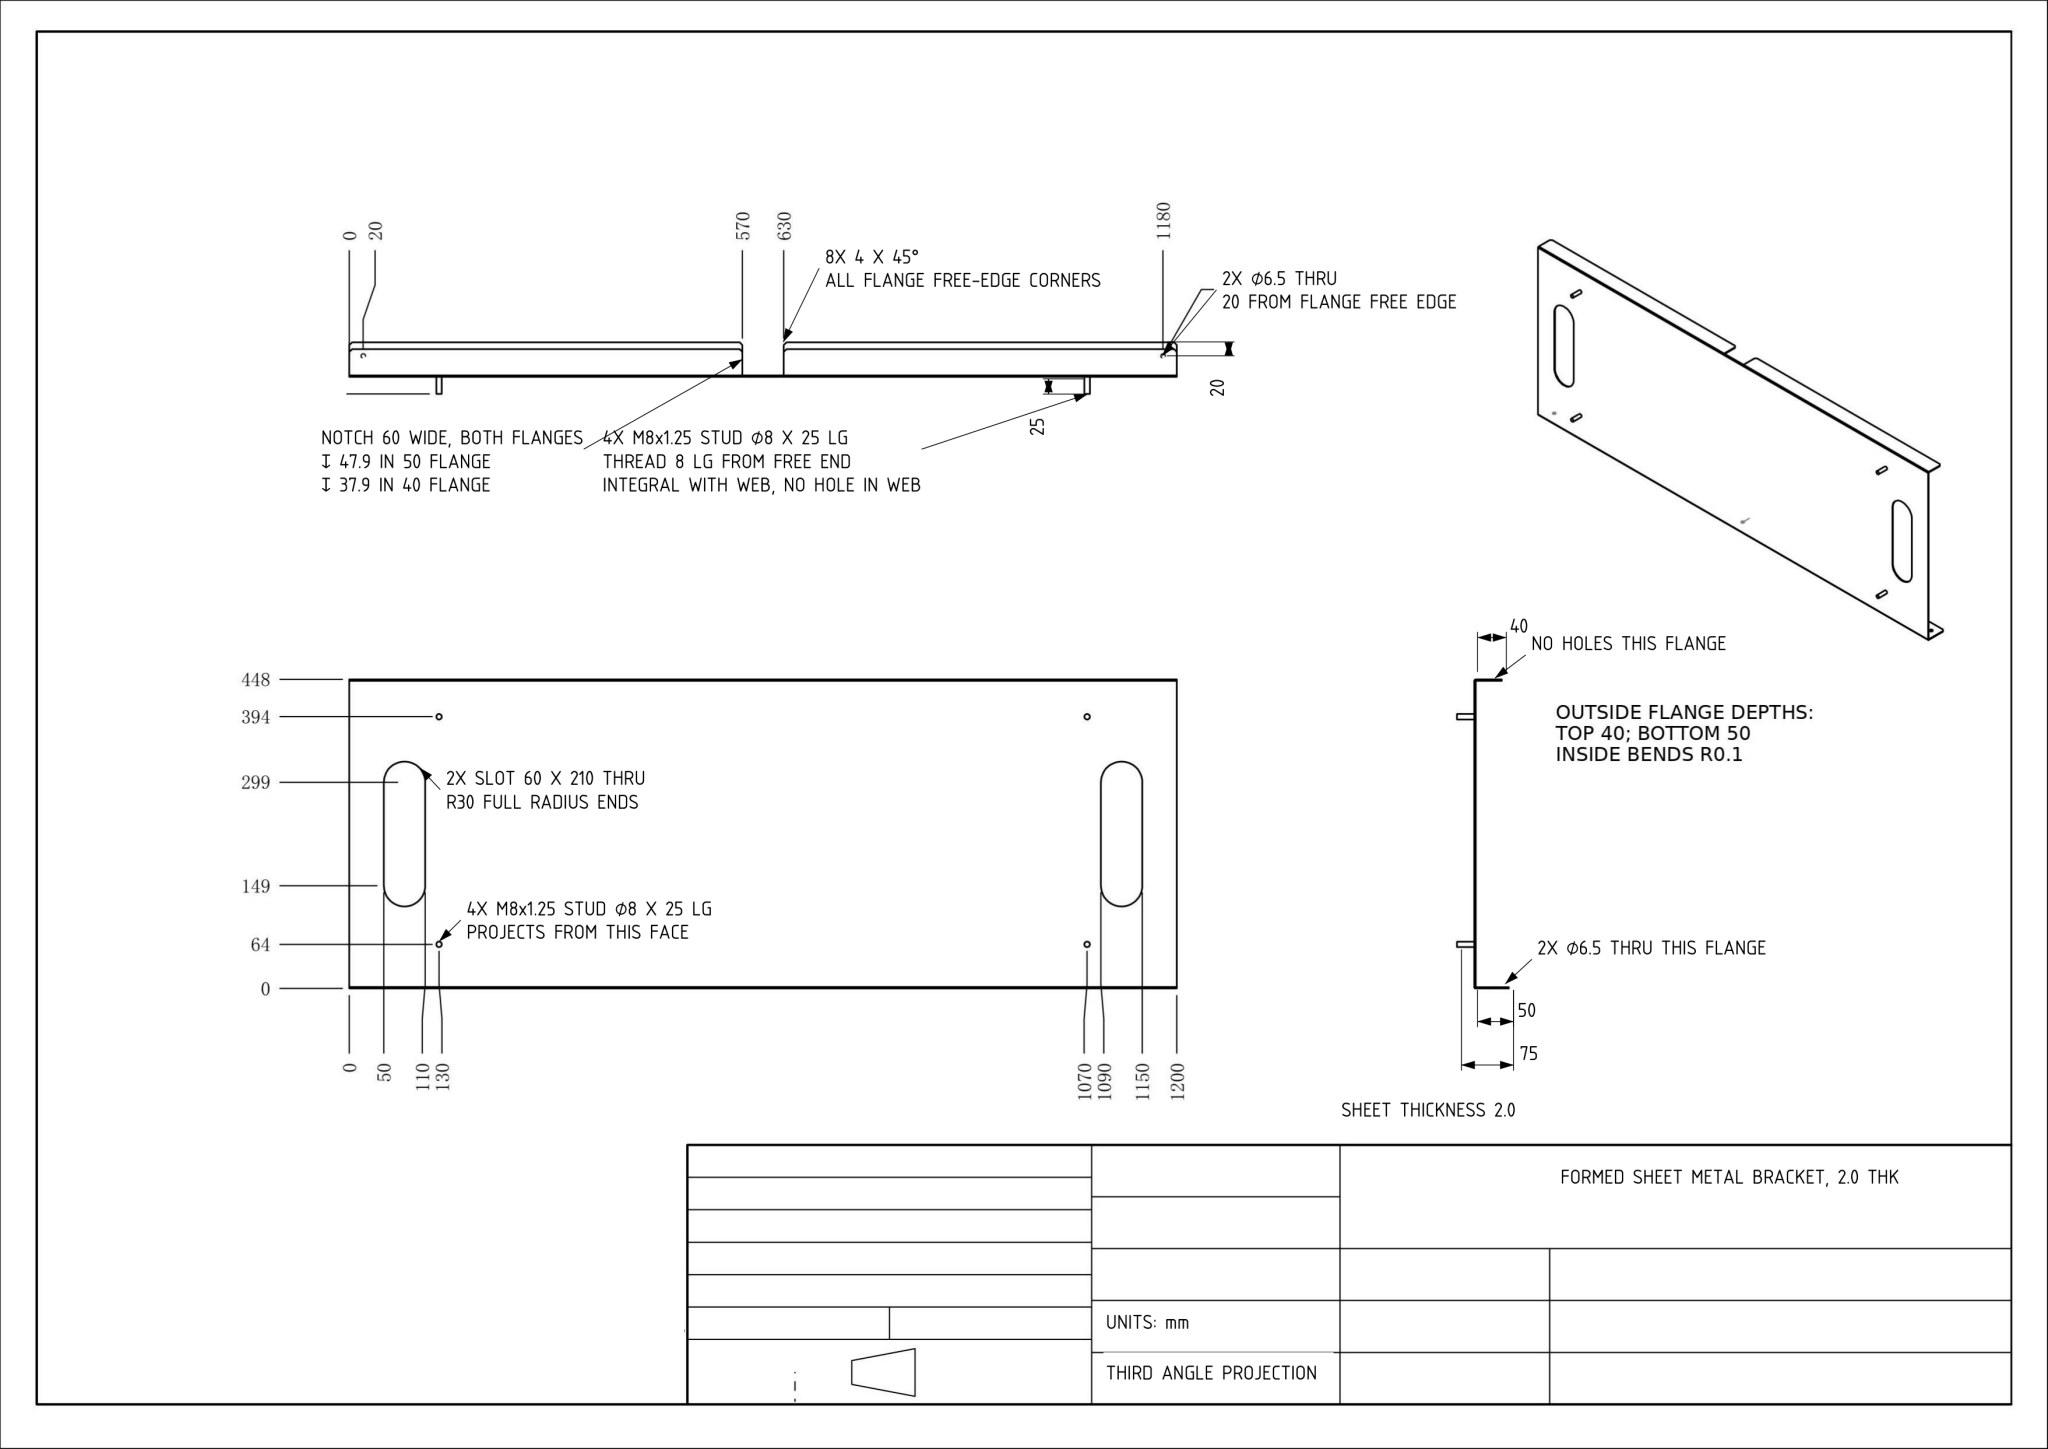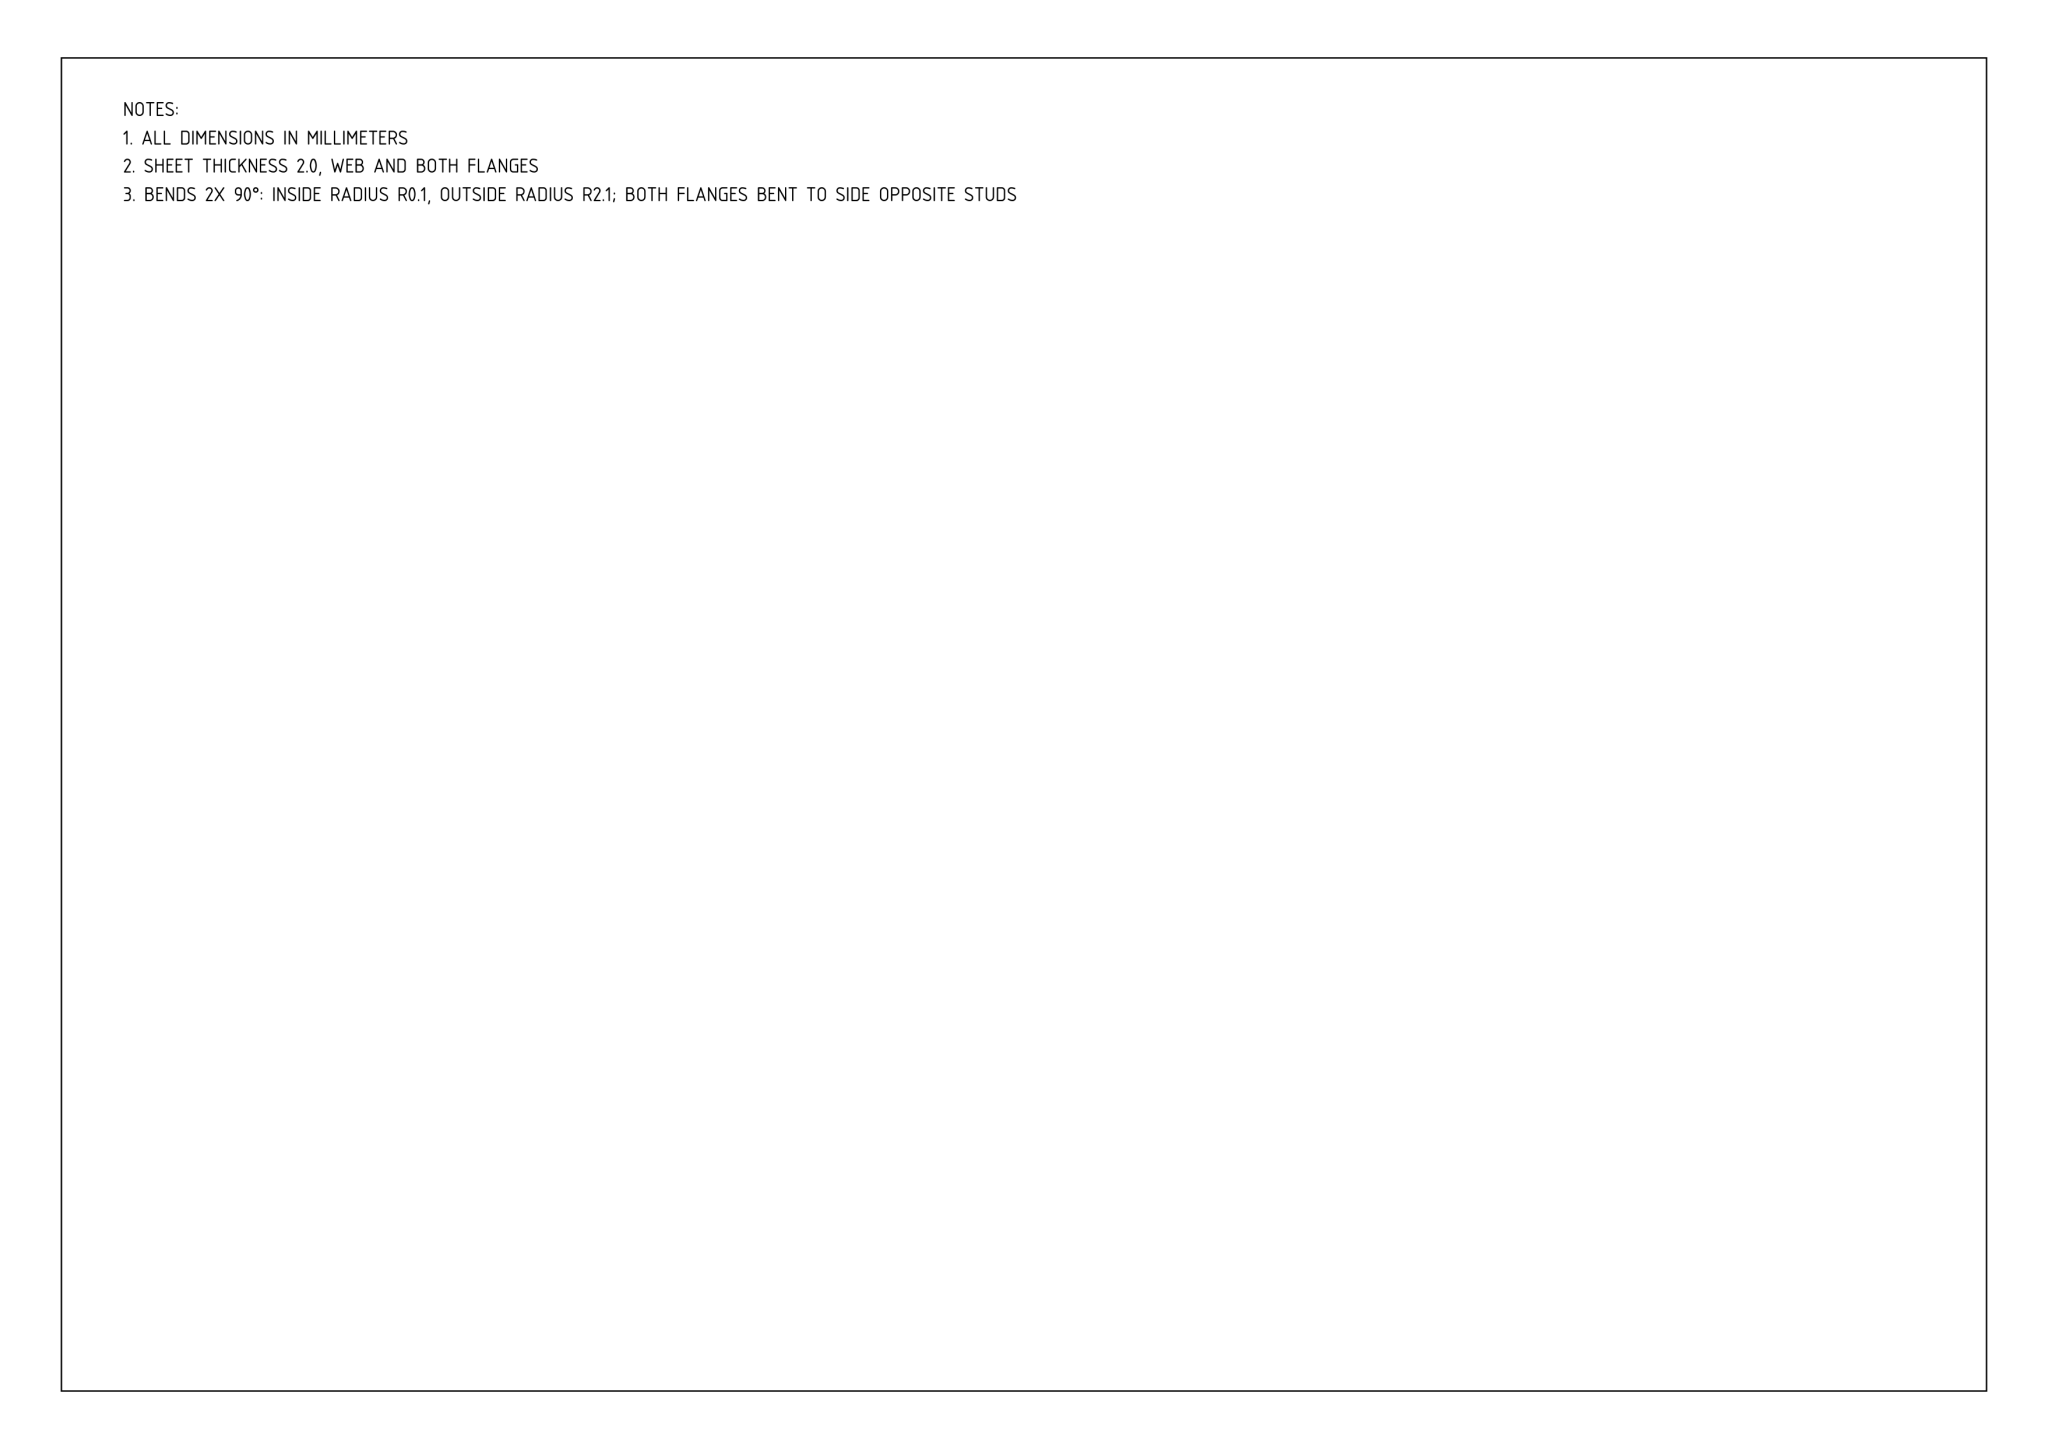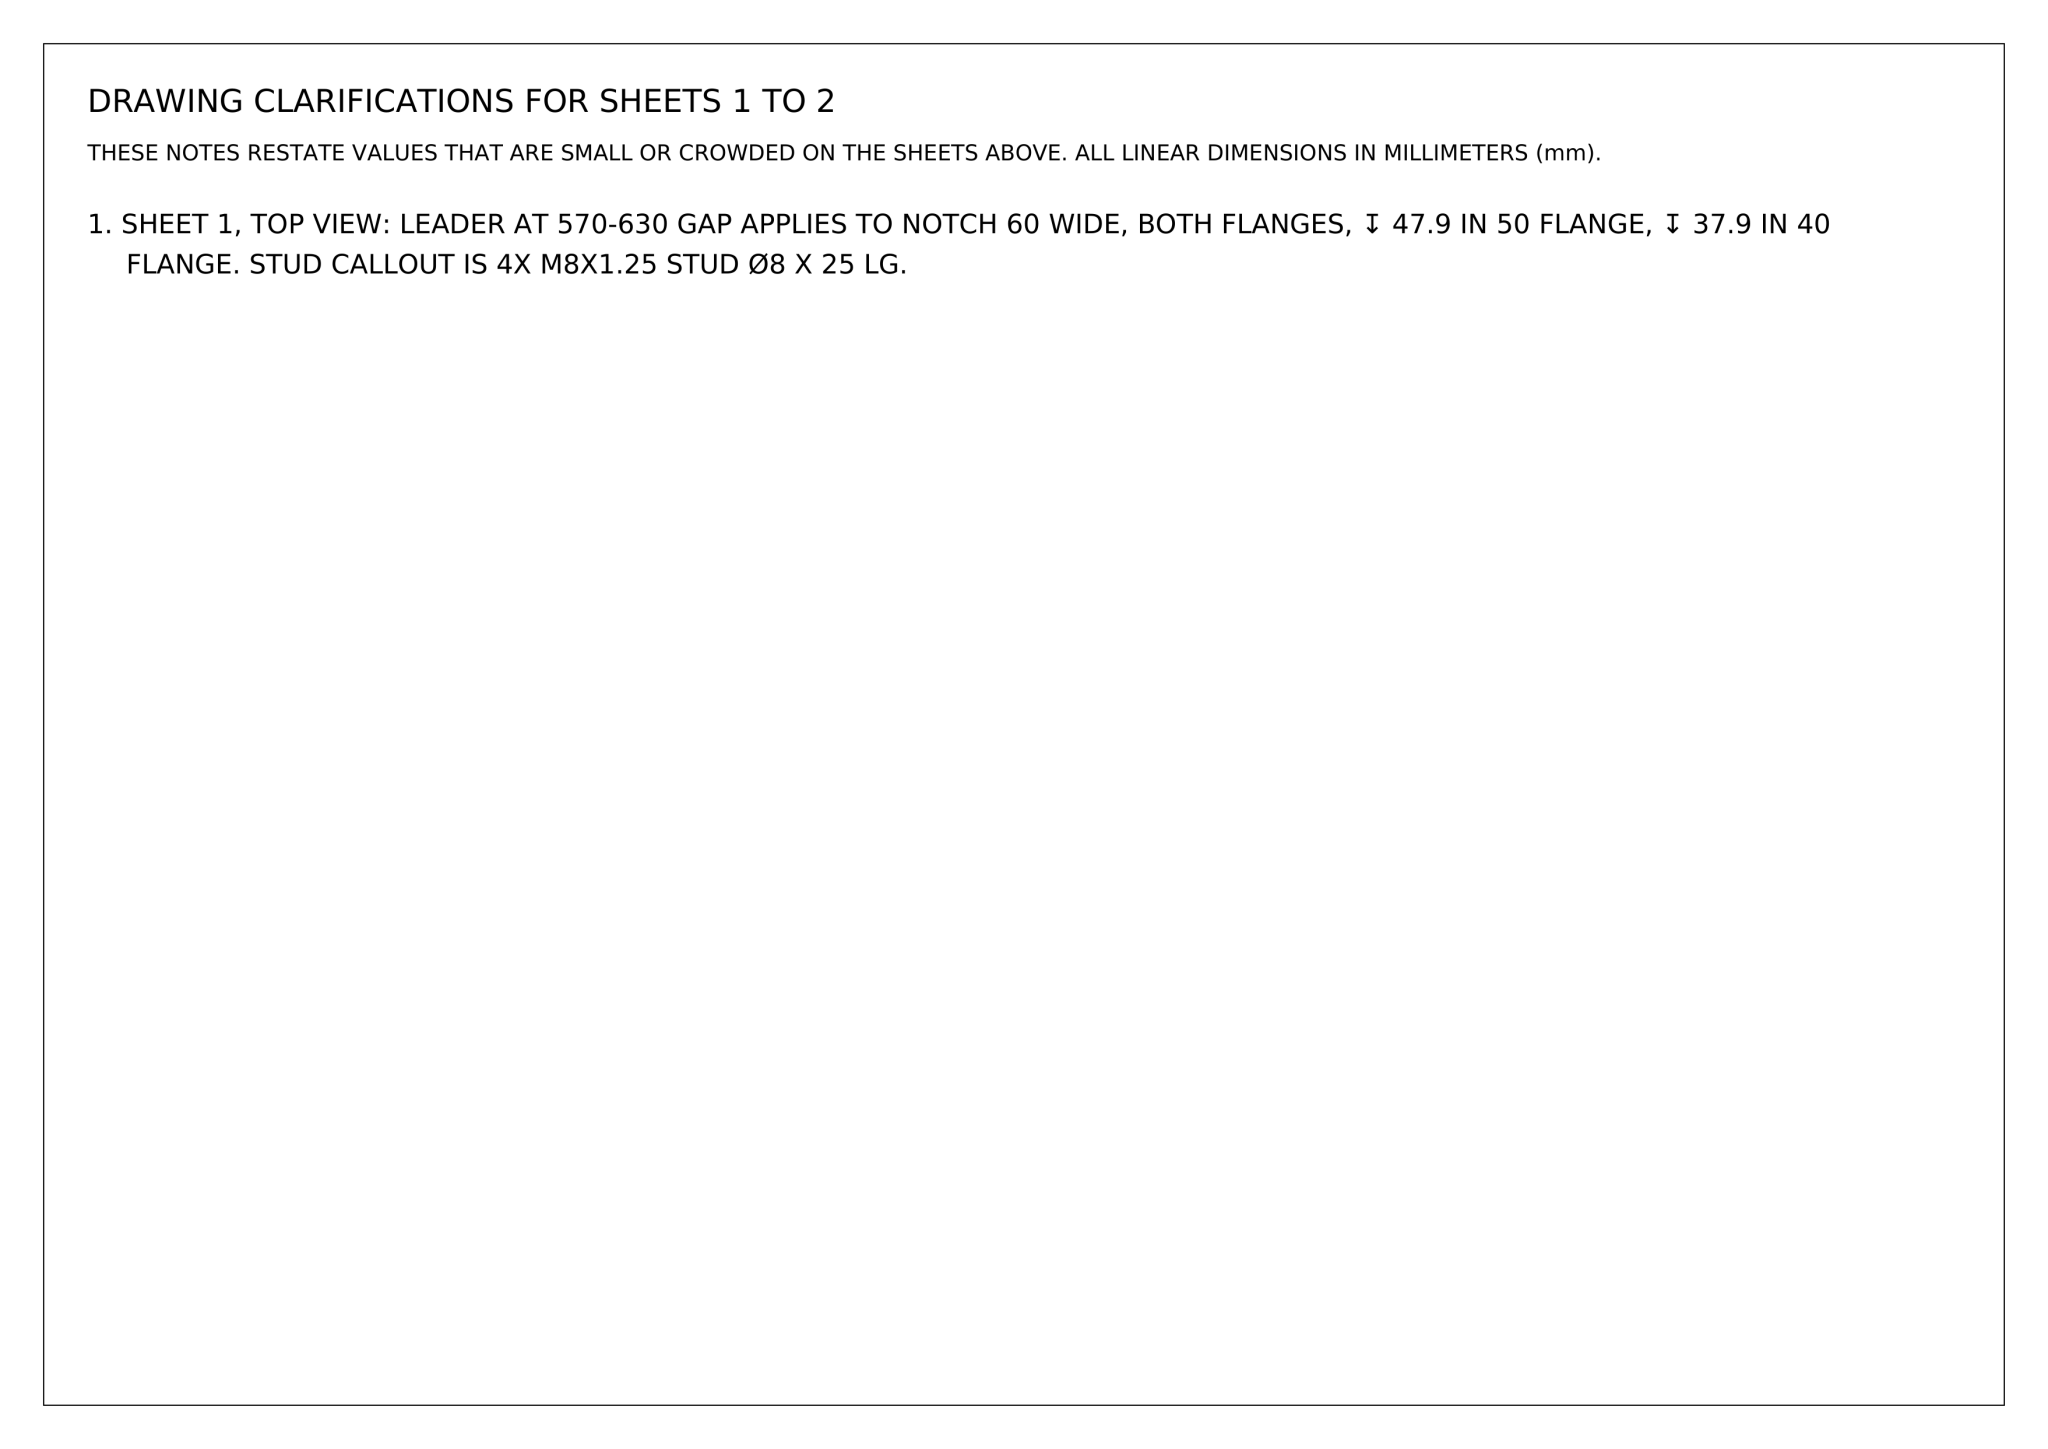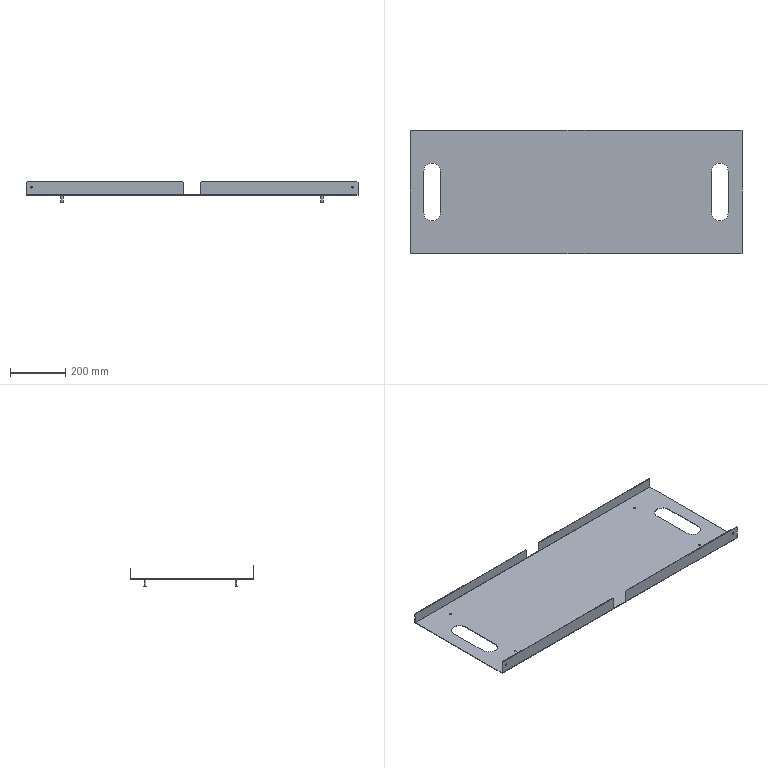Part | NX | mm | 1 solid | 66 faces | box 1200 x 448 x 75 mm | volume 1226494 mm3 | plane 46 | cylinder 20 | commonest cylinder face diameters 8 x8 6.5 x4 60 x4 4.2 x2 0.2 x2